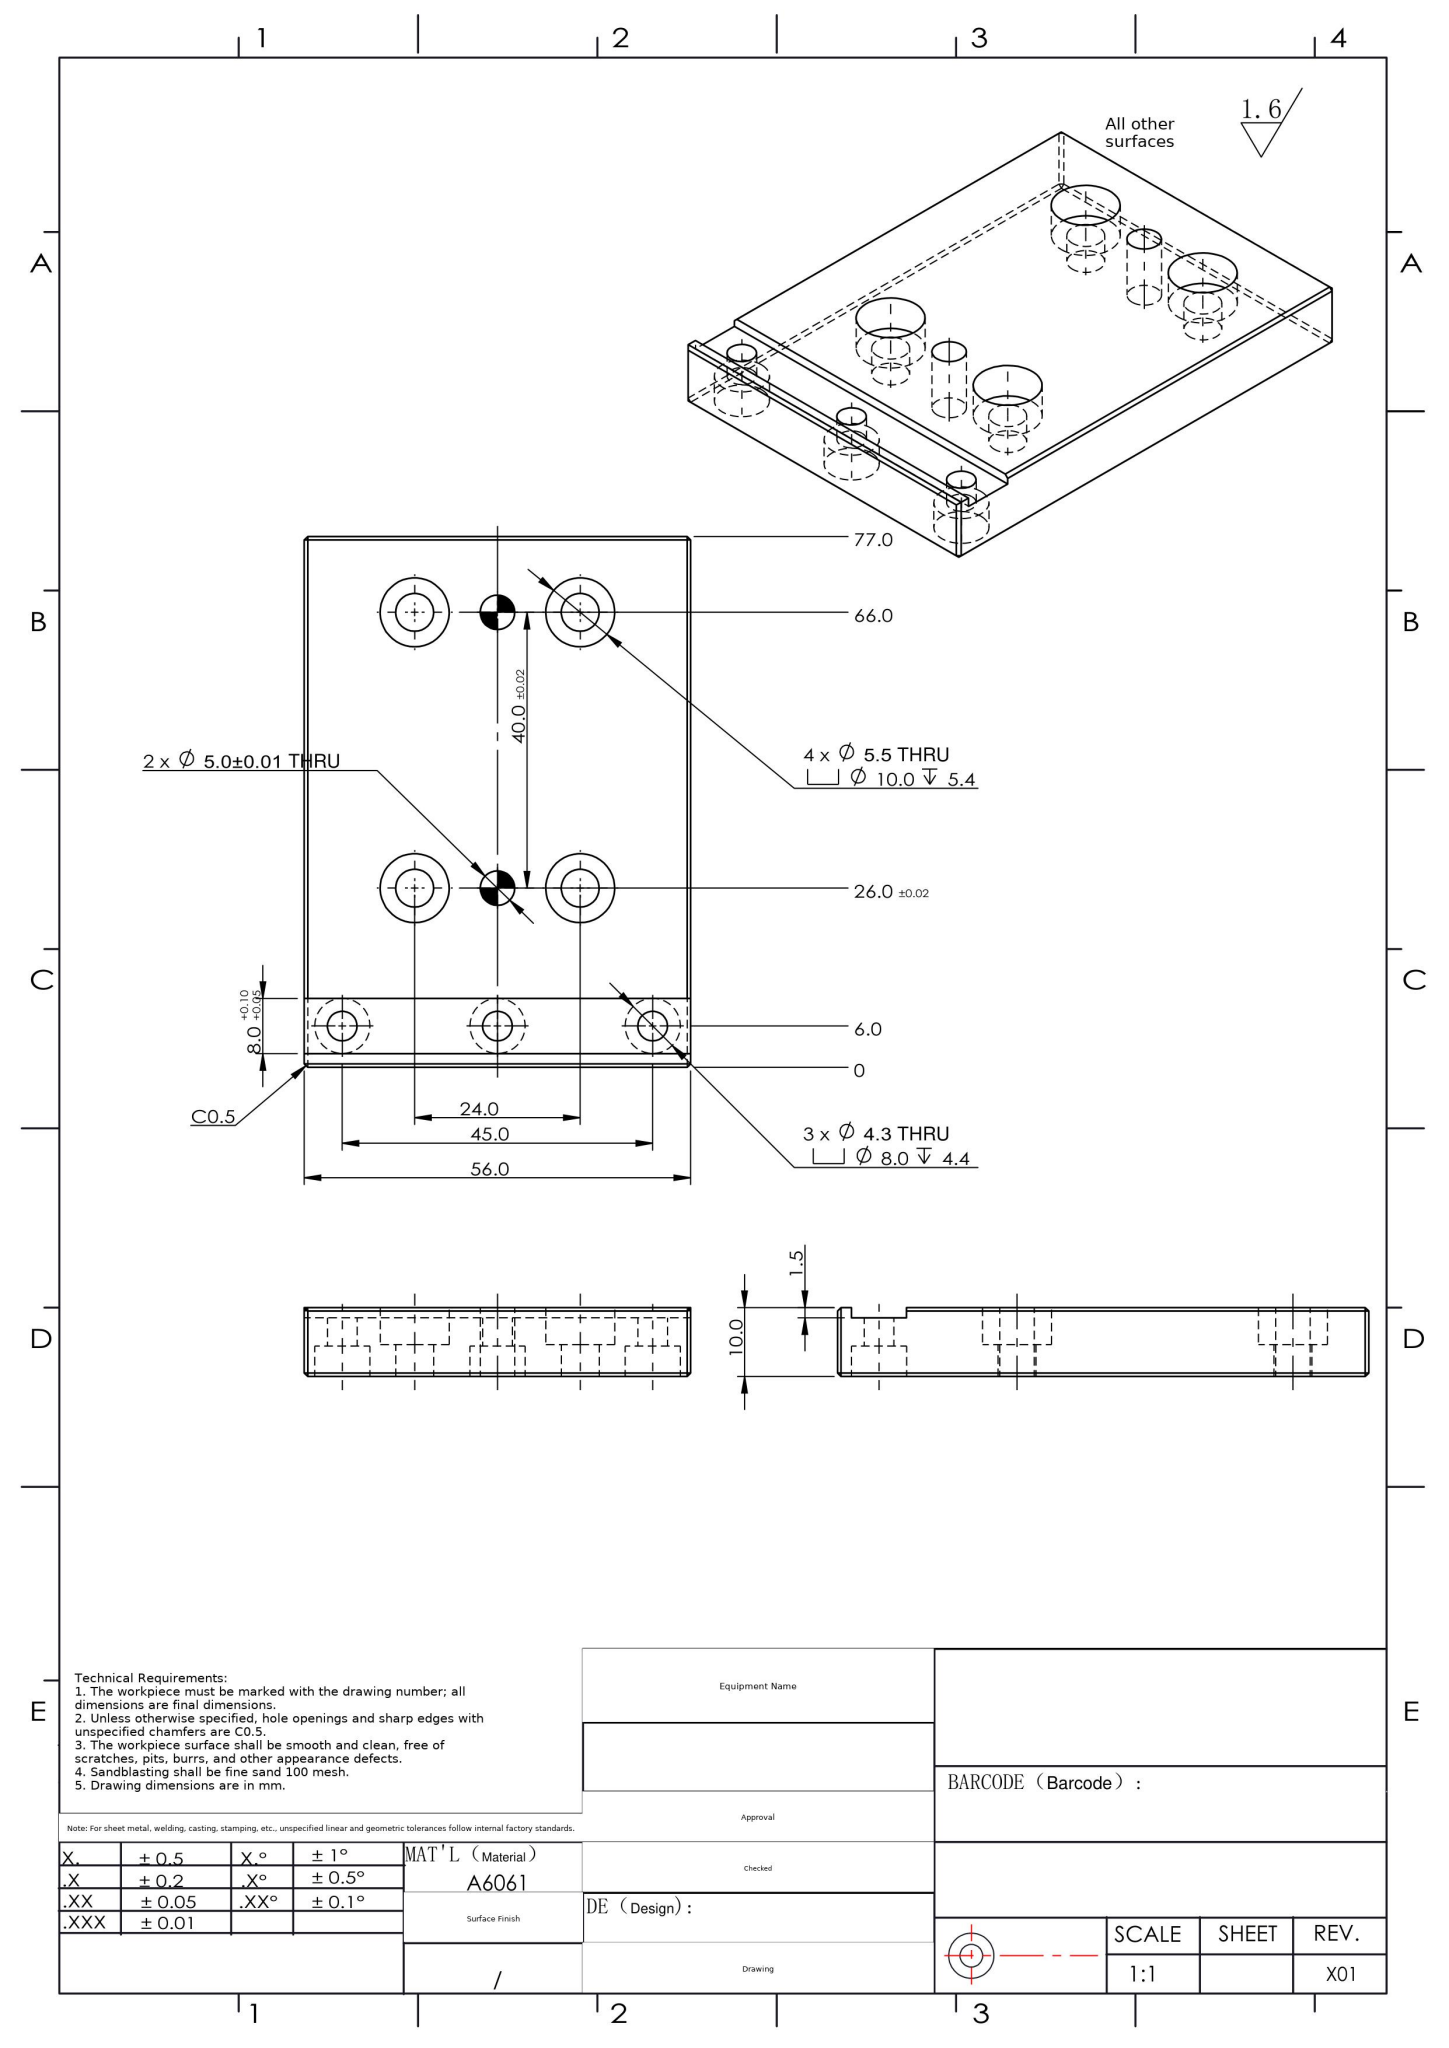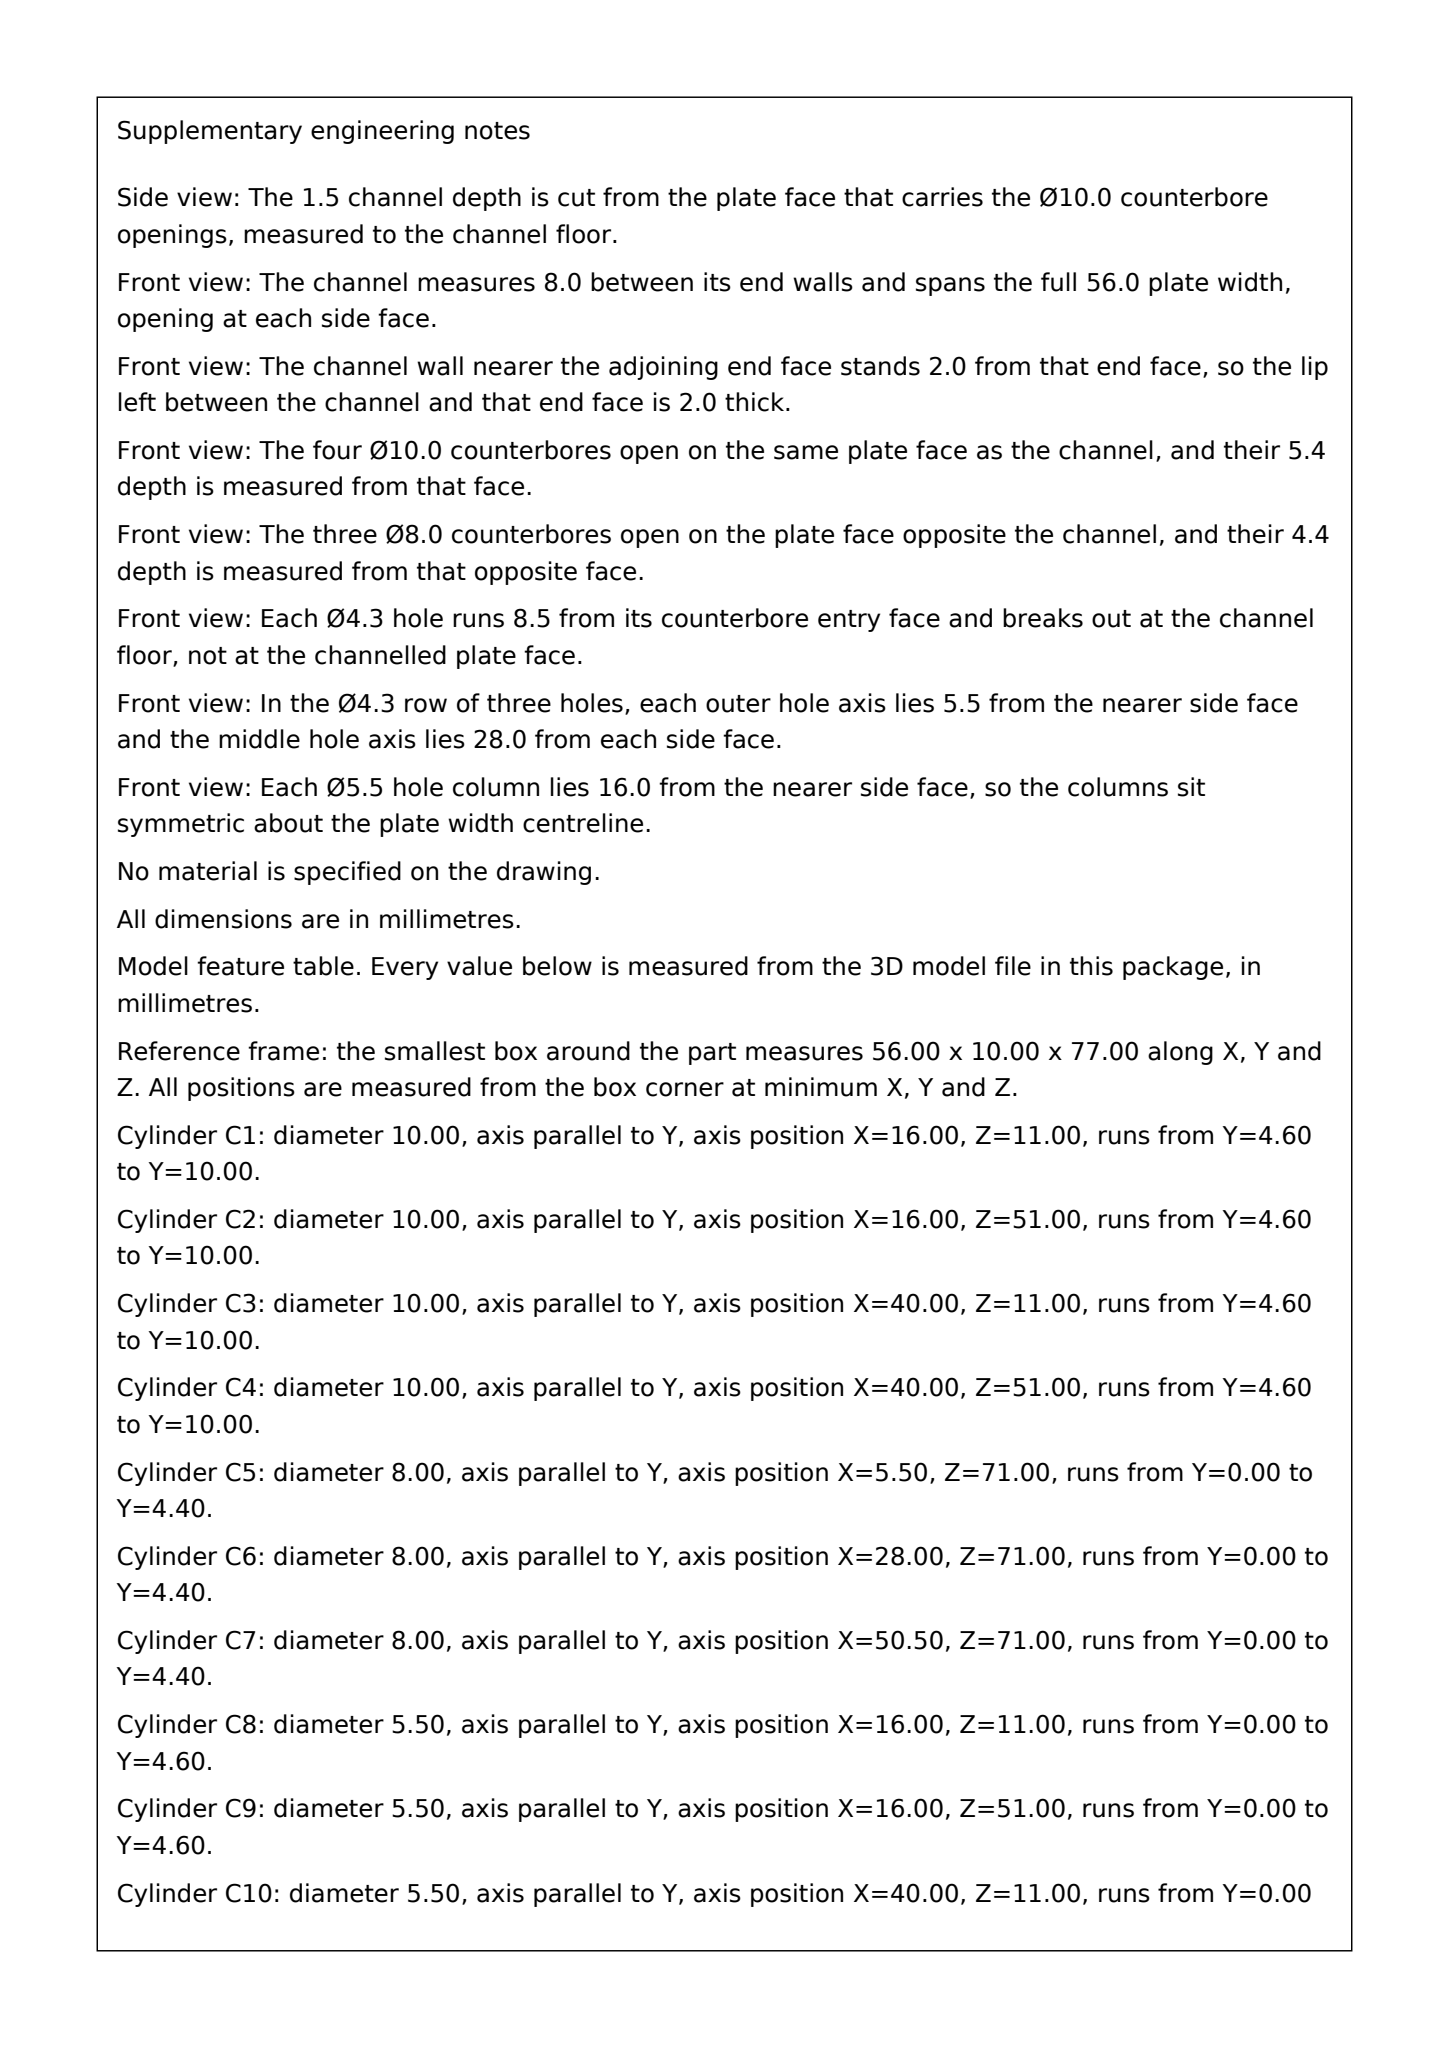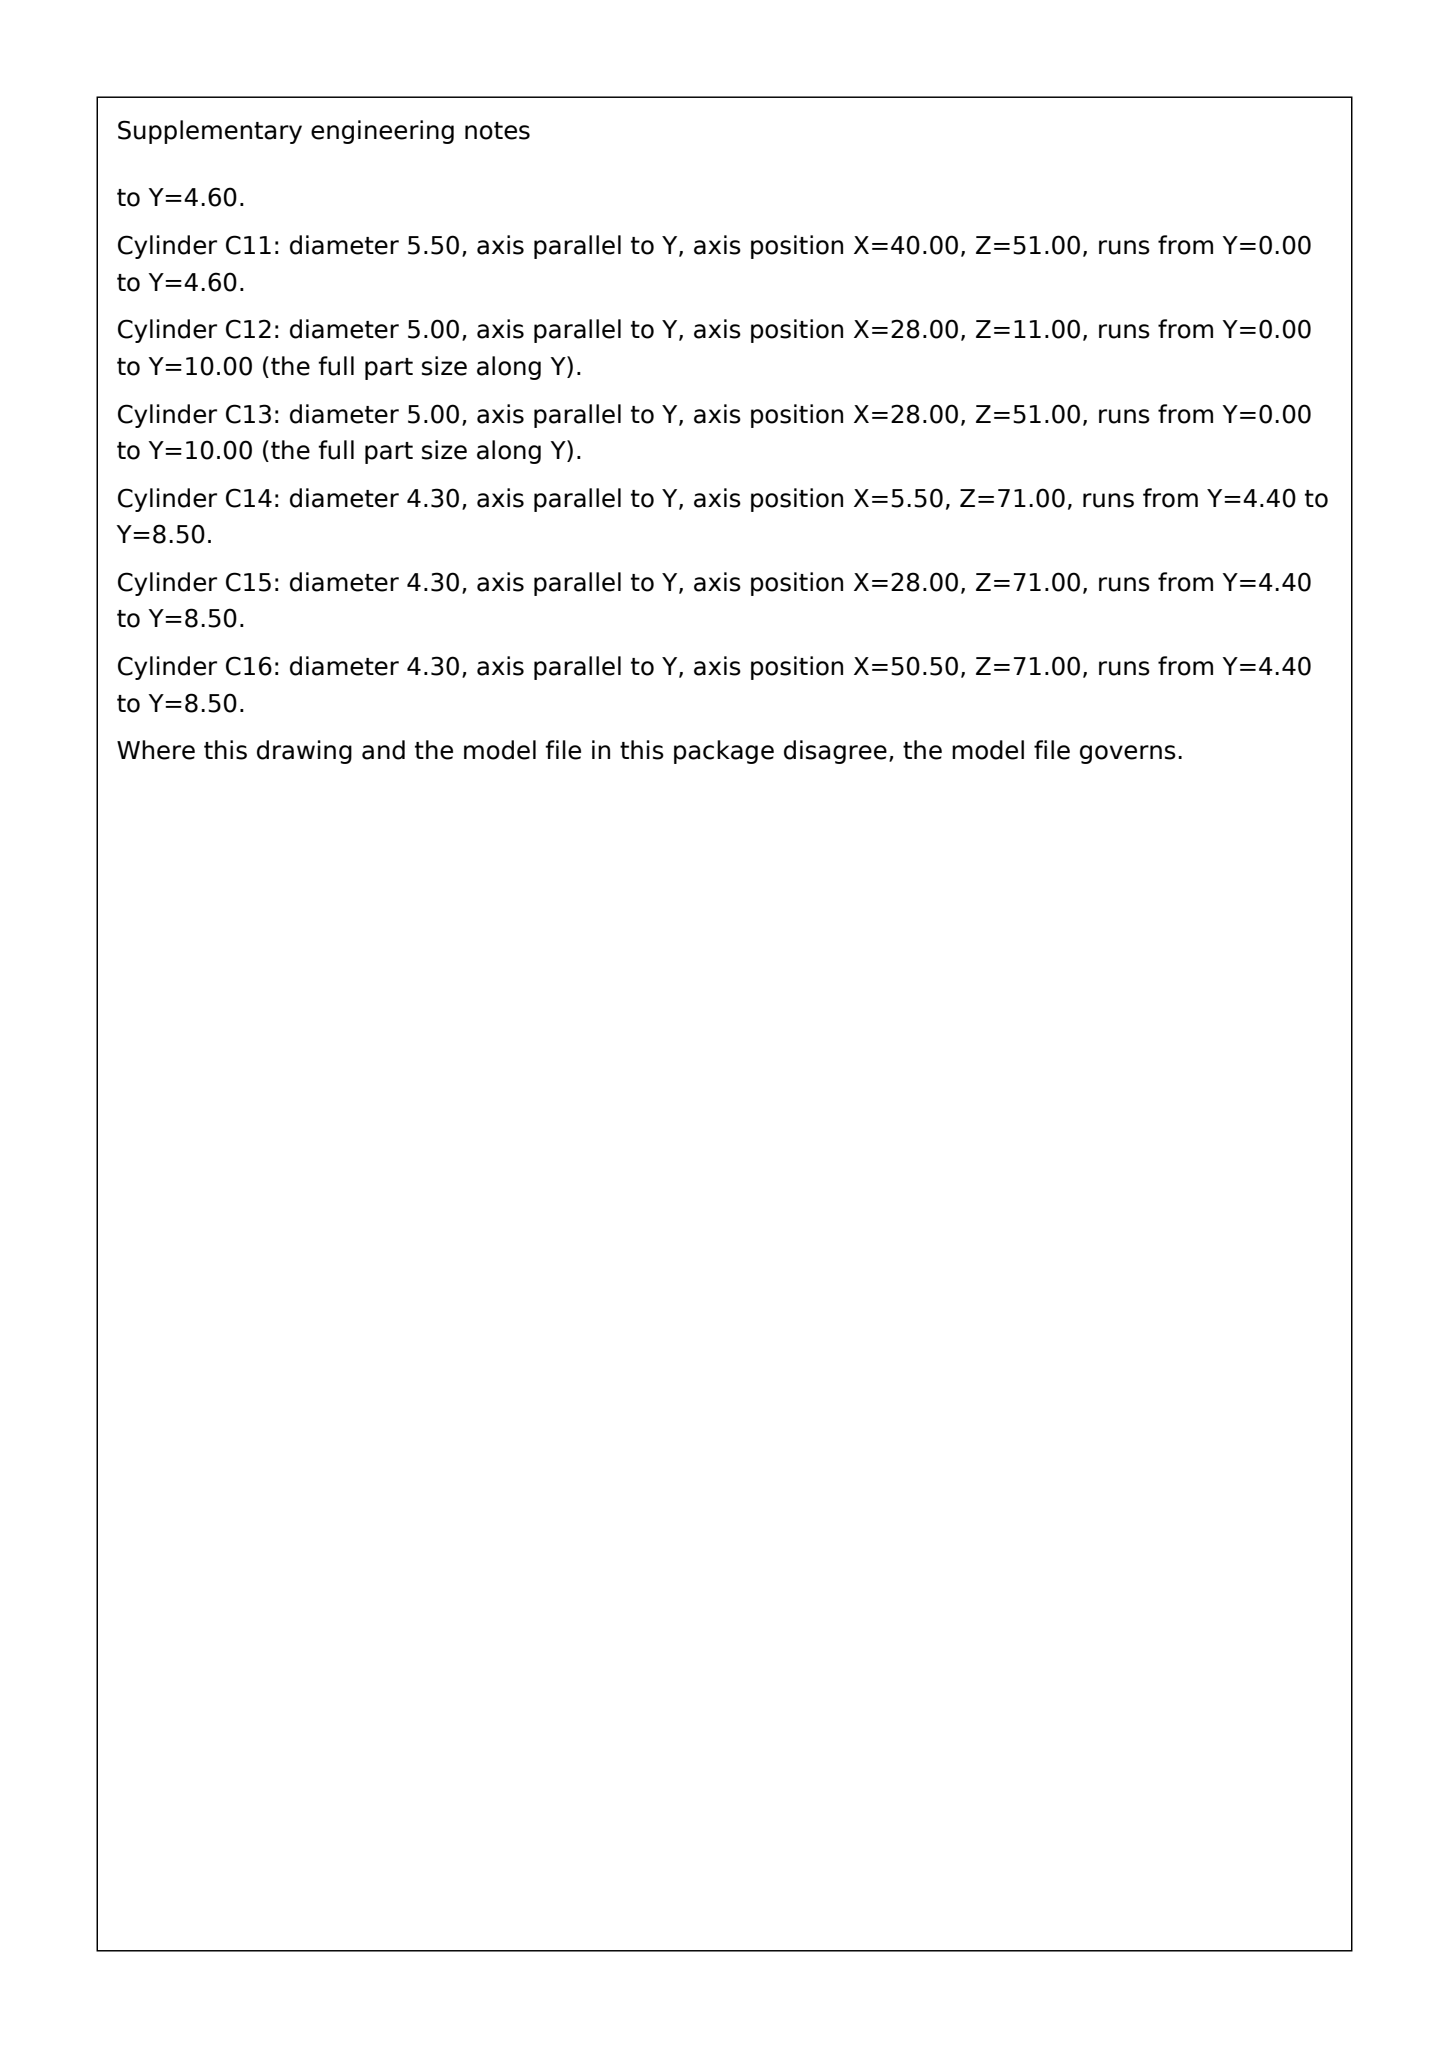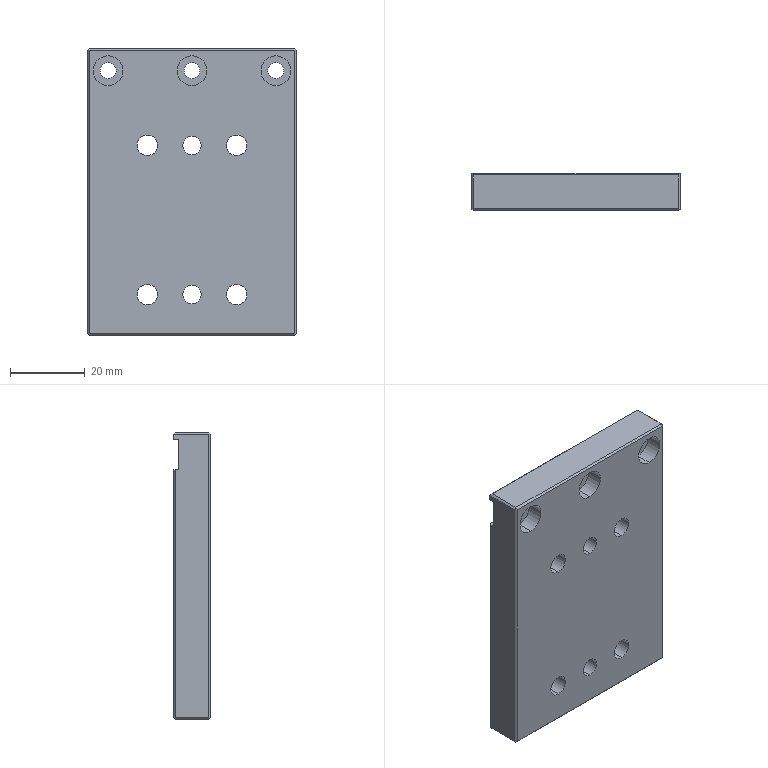Part | SolidWorks | mm | material A6061 | 1 solid | 67 faces | box 56 x 10 x 77 mm | volume 39011 mm3 | plane 35 | cylinder 32 | commonest cylinder face diameters 10 x8 5.5 x8 8 x6 4.3 x6 5 x4
Drawing notes:
① 2.0 = BTM EDGE TO 8.0 WIDE x 1.5 DP STEP, NOT A CHAMFER | from the solid: Z planes at 77.0 (btm edge in view), 75.0 and 67.0 give 2.0 land + 8.0 wide recess; Y planes 10.0 and 8.5 give 1.5 deep step
build123d program:
from build123d import *

# Parameters (mm, degrees)
SKETCH1_W                                       = 56
SKETCH1_H                                       = 10
BOSS_EXTRUDE1_DEPTH                             = 77
SKETCH3_W                                       = 56
SKETCH3_H                                       = 8
CUT_EXTRUDE1_DEPTH                              = 1.5
M4_HEX_SOCKET_HEAD_CAP_SCREW_CBORE1_D           = 4.3
M4_HEX_SOCKET_HEAD_CAP_SCREW_CBORE1_CBORE_D     = 8
M4_HEX_SOCKET_HEAD_CAP_SCREW_CBORE1_CBORE_DEPTH = 4.4
M5_HEX_SOCKET_HEAD_CAP_SCREW_CBORE1_D           = 5.5
M5_HEX_SOCKET_HEAD_CAP_SCREW_CBORE1_CBORE_D     = 10
M5_HEX_SOCKET_HEAD_CAP_SCREW_CBORE1_CBORE_DEPTH = 5.4
HOLE1_D                                         = 5
CHAMFER1_SIZE                                   = 0.5


with BuildPart() as part:
    # Sketch1 → Boss-Extrude1 (new body)
    with BuildSketch(Plane.XY):
        Rectangle(SKETCH1_W, SKETCH1_H)
    extrude(amount=BOSS_EXTRUDE1_DEPTH)

    # Sketch3 → Cut-Extrude1 (cut)
    with BuildSketch(Plane(origin=(0, 5, 0), x_dir=(1, 0, 0), z_dir=(0, 1, 0))):
        with Locations((0, -71)):
            Rectangle(SKETCH3_W, SKETCH3_H)
    extrude(amount=-CUT_EXTRUDE1_DEPTH, mode=Mode.SUBTRACT)

    # M4 Hex Socket Head Cap Screw CBORE1 (through all)
    with Locations(Plane(origin=(0, -5, 0), x_dir=(-1, 0, 0), z_dir=(0, -1, 0))):
        with Locations((22.5, -71), (0, -71), (-22.5, -71)):
            CounterBoreHole(M4_HEX_SOCKET_HEAD_CAP_SCREW_CBORE1_D / 2, M4_HEX_SOCKET_HEAD_CAP_SCREW_CBORE1_CBORE_D / 2, M4_HEX_SOCKET_HEAD_CAP_SCREW_CBORE1_CBORE_DEPTH)

    # M5 Hex Socket Head Cap Screw CBORE1 (through all)
    with Locations(Plane(origin=(0, 5, 0), x_dir=(1, 0, 0), z_dir=(0, 1, 0))):
        with Locations((12, -51), (-12, -51), (12, -11), (-12, -11)):
            CounterBoreHole(M5_HEX_SOCKET_HEAD_CAP_SCREW_CBORE1_D / 2, M5_HEX_SOCKET_HEAD_CAP_SCREW_CBORE1_CBORE_D / 2, M5_HEX_SOCKET_HEAD_CAP_SCREW_CBORE1_CBORE_DEPTH)

    # Hole1 (through all)
    with Locations(Plane(origin=(0, 5, 0), x_dir=(1, 0, 0), z_dir=(0, 1, 0))):
        with Locations((0, -11), (0, -51)):
            Hole(HOLE1_D / 2)

    # Chamfer1
    chamfer1_edges = [part.edges().sort_by_distance(p)[0] for p in [
        (0, -5, 77),
        (-28, 0, 77),
        (0, 5, 77),
        (28, 0, 77),
        (0, 5, 0),
        (-28, 5, 33.5),
        (-28, 0, 0),
        (28, 5, 33.5),
        (28, 0, 0),
        (28, -5, 38.5),
        (0, -5, 0),
        (-28, -5, 38.5),
    ]]
    chamfer(chamfer1_edges, length=CHAMFER1_SIZE)


solid = part.part